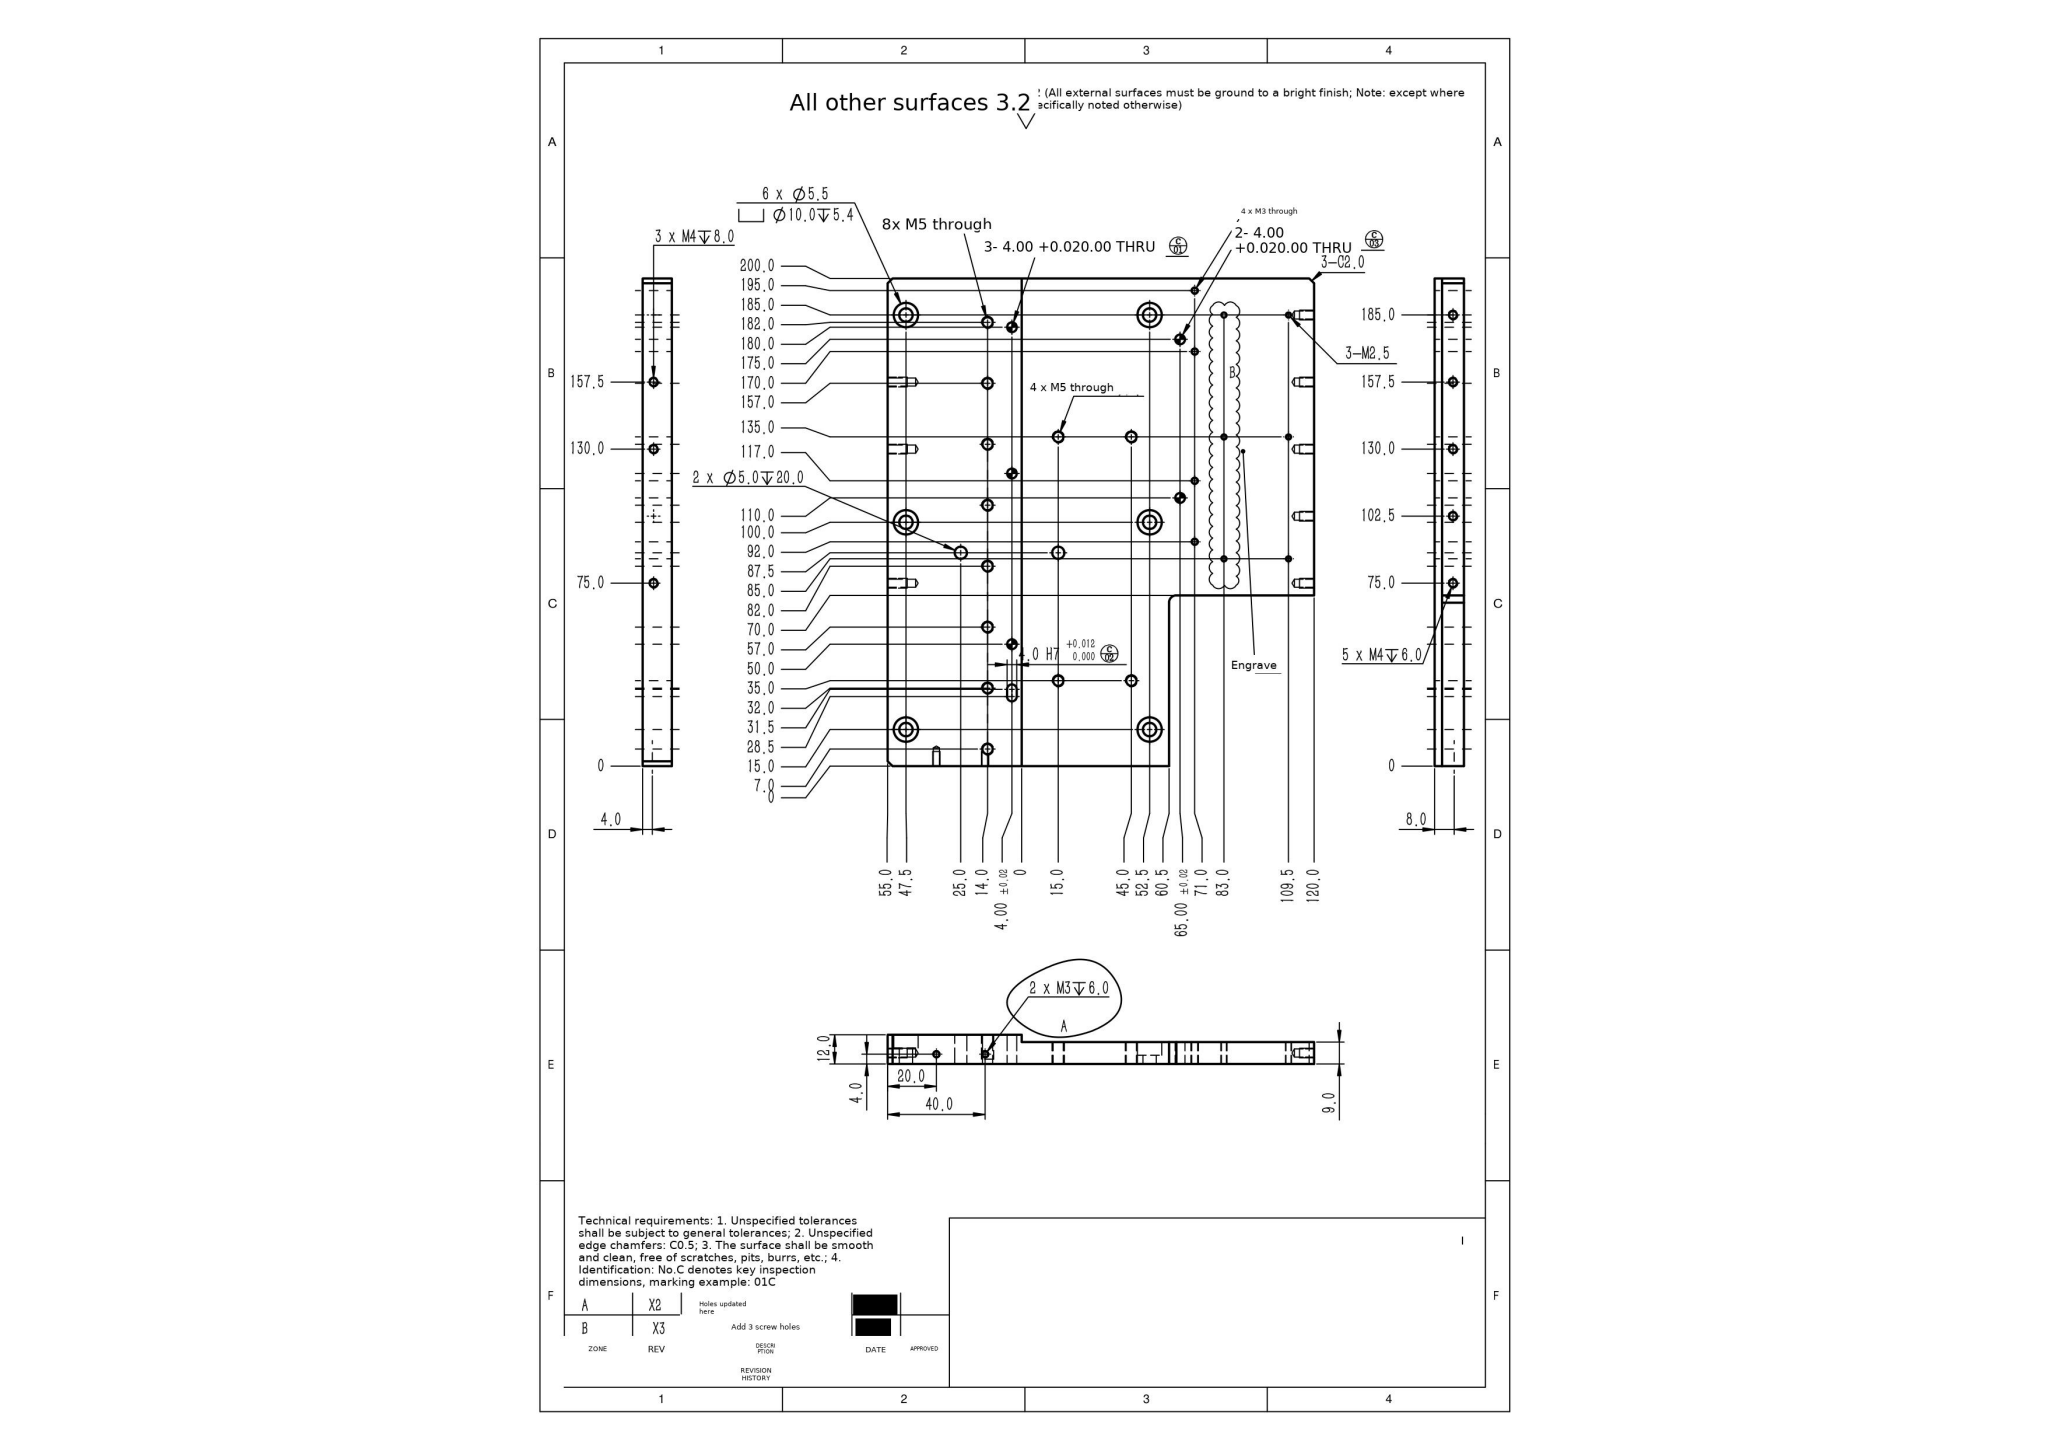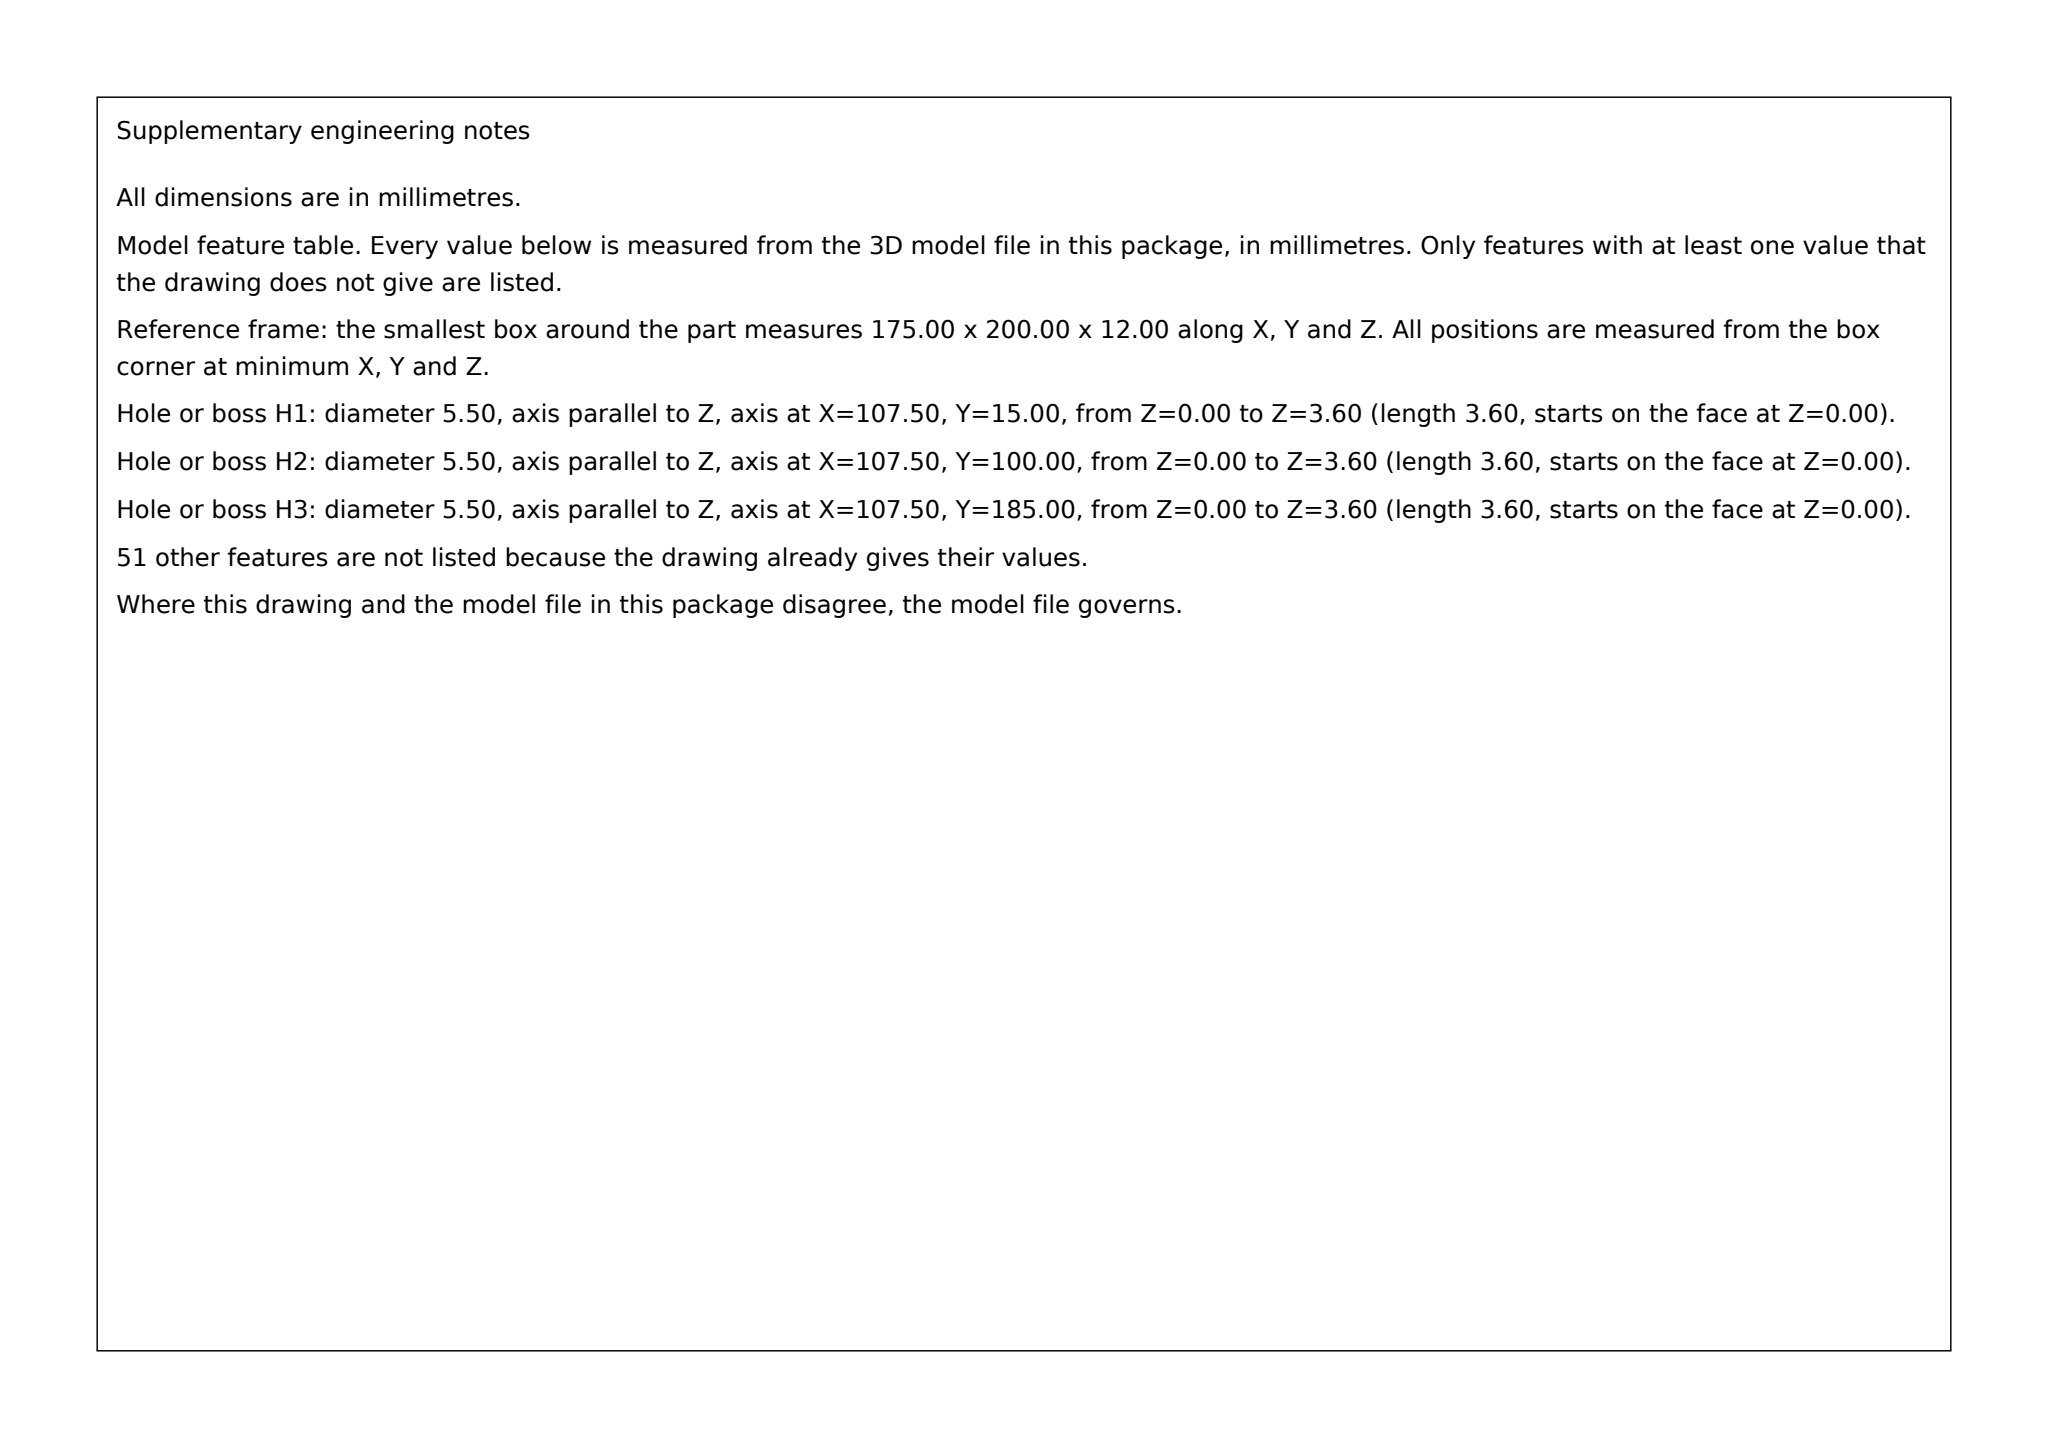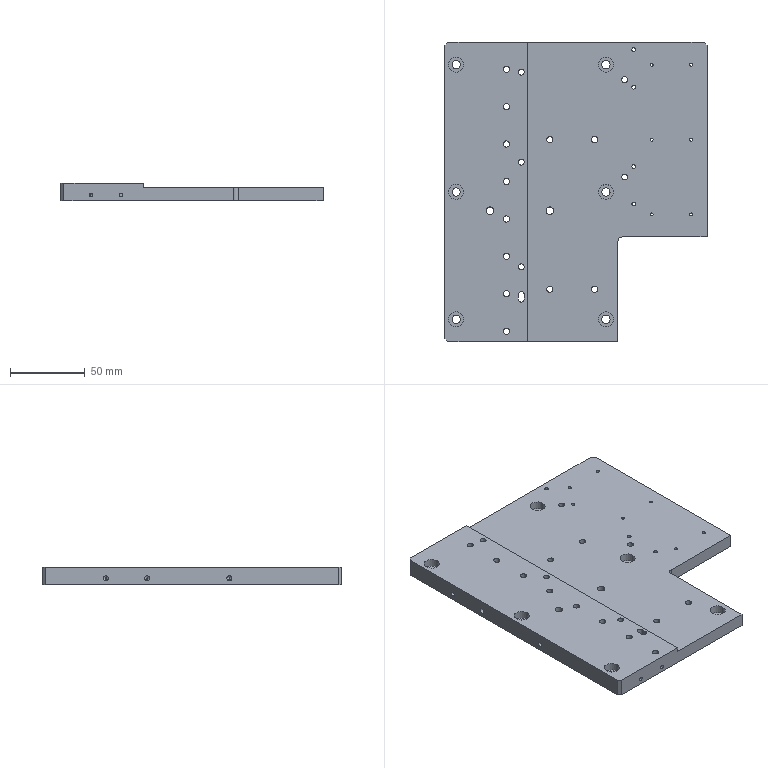Part | SolidWorks | mm | 1 solid | 145 faces | box 175 x 200 x 12 mm | volume 302897 mm3 | cylinder 105 | plane 21 | cone 19 | commonest cylinder face diameters 4.2 x24 3.3 x16 2.05 x12 2.5 x12 4 x12 10 x12 5.5 x12 5 x4
build123d program:
from build123d import *

# Parameters (mm, degrees)
SKETCH1_W                                       = 100
SKETCH1_H                                       = 150
BOSS_EXTRUDE1_DEPTH                             = 12
SKETCH2_W                                       = 60
SKETCH2_H                                       = 150
CUT_EXTRUDE1_DEPTH                              = 3
M5_TAPPED_HOLE2_D                               = 4.2
F_5_0_5_DIAMETER_HOLE1_D                        = 5
F_5_0_5_DIAMETER_HOLE1_DEPTH                    = 20
F_5_0_5_DIAMETER_HOLE1_TIP                      = 1.502
LPATTERN1_COUNT                                 = 6
LPATTERN1_PITCH                                 = 25
F_4_0_4_DIAMETER_HOLE1_D                        = 4
MOVE_FACE1_BY                                   = 15
MOVE_FACE2_BY                                   = 15
MOVE_FACE3_BY                                   = 50
M5_HEX_SOCKET_HEAD_CAP_SCREW_CBORE4_D           = 5.5
M5_HEX_SOCKET_HEAD_CAP_SCREW_CBORE4_CBORE_D     = 10
M5_HEX_SOCKET_HEAD_CAP_SCREW_CBORE4_CBORE_DEPTH = 5.4
M5_HEX_SOCKET_HEAD_CAP_SCREW_CBORE5_D           = 5.5
M5_HEX_SOCKET_HEAD_CAP_SCREW_CBORE5_CBORE_D     = 10
M5_HEX_SOCKET_HEAD_CAP_SCREW_CBORE5_CBORE_DEPTH = 5.4
CHAMFER1_SIZE                                   = 2
SKETCH23_R                                      = 2
CUT_EXTRUDE3_DEPTH                              = 232.017
SKETCH24_R                                      = 2
CUT_EXTRUDE4_DEPTH                              = 231.881
M3_TAPPED_HOLE1_D                               = 2.5
SKETCH27_W                                      = 9
SKETCH27_H                                      = 140
BOSS_EXTRUDE2_DEPTH                             = 45
M3_TAPPED_HOLE2_D                               = 2.5
M2_5_TAPPED_HOLE1_D                             = 2.05
FILLET1_R                                       = 3
M4_TAPPED_HOLE3_D                               = 3.3
M4_TAPPED_HOLE3_DEPTH                           = 8.1
M4_TAPPED_HOLE3_TIP                             = 0.9914
CHAMFER2_SIZE                                   = 2
M4_TAPPED_HOLE4_D                               = 3.3
M4_TAPPED_HOLE4_DEPTH                           = 11.5
M4_TAPPED_HOLE4_TIP                             = 0.9914
SKETCH40_W                                      = 30
SKETCH40_H                                      = 60
CUT_EXTRUDE5_DEPTH                              = 9
SKETCH41_W                                      = 59.5
SKETCH41_H                                      = 10
CUT_EXTRUDE6_DEPTH                              = 9
M5_TAPPED_HOLE3_D                               = 4.2
M5_TAPPED_HOLE3_DEPTH                           = 14
M5_TAPPED_HOLE3_TIP                             = 1.262
M3_TAPPED_HOLE3_D                               = 2.5
M3_TAPPED_HOLE3_DEPTH                           = 7.5
M3_TAPPED_HOLE3_TIP                             = 0.7511
LPATTERN3_COUNT                                 = 2
LPATTERN3_PITCH                                 = 26.5
FILLET2_R                                       = 3


with BuildPart() as part:
    # Sketch1 → Boss-Extrude1 (new body)
    with BuildSketch(Plane.XY):
        with Locations((50, 75)):
            Rectangle(SKETCH1_W, SKETCH1_H)
    extrude(amount=BOSS_EXTRUDE1_DEPTH)

    # Sketch2 → Cut-Extrude1 (cut)
    with BuildSketch(Plane.XY.offset(12)):
        with Locations((70, 75)):
            Rectangle(SKETCH2_W, SKETCH2_H)
    extrude(amount=-CUT_EXTRUDE1_DEPTH, mode=Mode.SUBTRACT)

    # Sketch3_2 → M5 Tapped Hole1 (revolve, cut)
    with BuildSketch(Plane(origin=(26, 132, 12), x_dir=(0, -1, 0), z_dir=(1, 0, 0))):
        Polygon((0, 0), (0, 15.262), (2.1, 14), (2.1, 0), align=None)
    m5_tapped_hole1 = revolve(axis=Axis((26, 132, 18.35), (0, 0, -1)), mode=Mode.SUBTRACT)

    # M5 Tapped Hole2 (through all)
    with Locations(Plane(origin=(0, 0, 0), x_dir=(-1, 0, 0), z_dir=(0, 0, -1))):
        with Locations((-85, 35), (-55, 35), (-85, 135), (-55, 135)):
            Hole(M5_TAPPED_HOLE2_D / 2)

    # 5.0 _5_ Diameter Hole1
    with Locations(Plane(origin=(0, 0, 0), x_dir=(-1, 0, 0), z_dir=(0, 0, -1))):
        with Locations((-55, 87.5), (-15, 87.5)):
            Hole(F_5_0_5_DIAMETER_HOLE1_D / 2, depth=F_5_0_5_DIAMETER_HOLE1_DEPTH)
            with Locations((0, 0, -(F_5_0_5_DIAMETER_HOLE1_DEPTH + F_5_0_5_DIAMETER_HOLE1_TIP / 2))):  # 118° drill point
                Cone(0, F_5_0_5_DIAMETER_HOLE1_D / 2, F_5_0_5_DIAMETER_HOLE1_TIP, mode=Mode.SUBTRACT)

    # LPattern1: M5 Tapped Hole1 ×6
    with Locations(*[(0, -i * LPATTERN1_PITCH, 0) for i in range(1, LPATTERN1_COUNT)]):
        add(m5_tapped_hole1, mode=Mode.SUBTRACT)

    # 4.0 _4_ Diameter Hole1 (through all)
    with Locations(Plane(origin=(-0.2203, 3.564, 12), x_dir=(1, 0, 0), z_dir=(0, 0, 1))):
        with Locations((36.22, 116.436), (36.22, 46.436)):
            Hole(F_4_0_4_DIAMETER_HOLE1_D / 2)

    # Move Face1: a face moved outward by 15.0
    extrude(part.faces().sort_by_distance((100, 75, 4.5))[0], amount=MOVE_FACE1_BY, dir=(1, 0, 0))

    # Move Face2: a face moved outward by 15.0
    extrude(part.faces().sort_by_distance((0, 75, 6))[0], amount=MOVE_FACE2_BY, dir=(-1, 0, 0))

    # Move Face3: a face moved outward by 50.0
    extrude(part.faces().sort_by_distance((45.365, 150, 5.242))[0], amount=MOVE_FACE3_BY, dir=(0, 1, 0))

    # M5 Hex Socket Head Cap Screw CBORE4 (through all)
    with Locations(Plane.XY.offset(9)):
        with Locations((92.5, 185), (92.5, 100), (92.5, 15)):
            CounterBoreHole(M5_HEX_SOCKET_HEAD_CAP_SCREW_CBORE4_D / 2, M5_HEX_SOCKET_HEAD_CAP_SCREW_CBORE4_CBORE_D / 2, M5_HEX_SOCKET_HEAD_CAP_SCREW_CBORE4_CBORE_DEPTH)

    # M5 Hex Socket Head Cap Screw CBORE5 (through all)
    with Locations(Plane.XY.offset(12)):
        with Locations((-7.5, 185), (-7.5, 100), (-7.5, 15)):
            CounterBoreHole(M5_HEX_SOCKET_HEAD_CAP_SCREW_CBORE5_D / 2, M5_HEX_SOCKET_HEAD_CAP_SCREW_CBORE5_CBORE_D / 2, M5_HEX_SOCKET_HEAD_CAP_SCREW_CBORE5_CBORE_DEPTH)

    # Chamfer1
    chamfer1_edges = [part.edges().sort_by_distance(p)[0] for p in [
        (-15, 200, 6),
        (-15, 0, 6),
    ]]
    chamfer(chamfer1_edges, length=CHAMFER1_SIZE)

    # Sketch23 → Cut-Extrude3 (cut, through all)
    with BuildSketch(Plane.XY.offset(12)):
        with Locations((36, 180)):
            Circle(SKETCH23_R)
        with BuildLine():
            Line((38, 31.5), (38, 28.5))
            ThreePointArc((38, 28.5), (36, 26.5), (34, 28.5))
            Line((34, 28.5), (34, 31.5))
            ThreePointArc((34, 31.5), (36, 33.5), (38, 31.5))
        make_face()
    extrude(amount=-CUT_EXTRUDE3_DEPTH, mode=Mode.SUBTRACT)

    # Sketch24 → Cut-Extrude4 (cut, through all)
    with BuildSketch(Plane.XY.offset(9)):
        with Locations((105, 175)):
            Circle(SKETCH24_R)
        with Locations((105, 110)):
            Circle(SKETCH24_R)
    extrude(amount=-CUT_EXTRUDE4_DEPTH, mode=Mode.SUBTRACT)

    # M3 Tapped Hole1 (through all)
    with Locations(Plane.XY.offset(9)):
        with Locations((111, 195), (111, 117)):
            Hole(M3_TAPPED_HOLE1_D / 2)

    # Sketch27 → Boss-Extrude2 (add)
    with BuildSketch(Plane(origin=(115, 0, 0), x_dir=(0, 0, -1), z_dir=(1, 0, 0))):
        with Locations((-4.5, 130)):
            Rectangle(SKETCH27_W, SKETCH27_H)
    extrude(amount=BOSS_EXTRUDE2_DEPTH)

    # M3 Tapped Hole2 (through all)
    with Locations(Plane.XY.offset(9)):
        with Locations((111, 170), (111, 92)):
            Hole(M3_TAPPED_HOLE2_D / 2)

    # M2.5 Tapped Hole1 (through all)
    with Locations(Plane.XY.offset(9)):
        with Locations((149.5, 185), (149.5, 85), (149.5, 135)):
            m2_5_tapped_hole1 = Hole(M2_5_TAPPED_HOLE1_D / 2)

    # Fillet1
    fillet1_edges = [part.edges().sort_by_distance(p)[0] for p in [
        (115, 60, 4.5),
    ]]
    fillet(fillet1_edges, radius=FILLET1_R)

    # M4 Tapped Hole3
    with Locations(Plane(origin=(160, 0, 0), x_dir=(0, 0, -1), z_dir=(1, 0, 0))):
        with Locations((-4.5, 185), (-4.5, 130), (-4.5, 75), (-4.5, 157.5), (-4.5, 102.5)):
            Hole(M4_TAPPED_HOLE3_D / 2, depth=M4_TAPPED_HOLE3_DEPTH)
            with Locations((0, 0, -(M4_TAPPED_HOLE3_DEPTH + M4_TAPPED_HOLE3_TIP / 2))):  # 118° drill point
                Cone(0, M4_TAPPED_HOLE3_D / 2, M4_TAPPED_HOLE3_TIP, mode=Mode.SUBTRACT)

    # Chamfer2
    chamfer2_edges = [part.edges().sort_by_distance(p)[0] for p in [
        (160, 200, 4.5),
        (160, 60, 4.5),
        (115, 0, 4.5),
    ]]
    chamfer(chamfer2_edges, length=CHAMFER2_SIZE)

    # M4 Tapped Hole4
    with Locations(Plane.ZY.offset(15)):
        with Locations((4.5, 157.5), (4.5, 130), (4.5, 75)):
            Hole(M4_TAPPED_HOLE4_D / 2, depth=M4_TAPPED_HOLE4_DEPTH)
            with Locations((0, 0, -(M4_TAPPED_HOLE4_DEPTH + M4_TAPPED_HOLE4_TIP / 2))):  # 118° drill point
                Cone(0, M4_TAPPED_HOLE4_D / 2, M4_TAPPED_HOLE4_TIP, mode=Mode.SUBTRACT)

    # Sketch40 → Cut-Extrude5 (cut)
    with BuildSketch(Plane.XY.offset(9)):
        with Locations((115.5, 30)):
            Rectangle(SKETCH40_W, SKETCH40_H)
    extrude(amount=-CUT_EXTRUDE5_DEPTH, mode=Mode.SUBTRACT)

    # Sketch41 → Cut-Extrude6 (cut)
    with BuildSketch(Plane.XY.offset(9)):
        with Locations((130.25, 65)):
            Rectangle(SKETCH41_W, SKETCH41_H)
    extrude(amount=-CUT_EXTRUDE6_DEPTH, mode=Mode.SUBTRACT)

    # M5 Tapped Hole3
    with Locations(Plane.XY.offset(12)):
        with Locations((26, 182), (26, 157)):
            Hole(M5_TAPPED_HOLE3_D / 2, depth=M5_TAPPED_HOLE3_DEPTH)
            with Locations((0, 0, -(M5_TAPPED_HOLE3_DEPTH + M5_TAPPED_HOLE3_TIP / 2))):  # 118° drill point
                Cone(0, M5_TAPPED_HOLE3_D / 2, M5_TAPPED_HOLE3_TIP, mode=Mode.SUBTRACT)

    # M3 Tapped Hole3
    with Locations(Plane(origin=(0, 0, 0), x_dir=(-1, 0, 0), z_dir=(0, -1, 0))):
        with Locations((-5, -4), (-25, -4)):
            Hole(M3_TAPPED_HOLE3_D / 2, depth=M3_TAPPED_HOLE3_DEPTH)
            with Locations((0, 0, -(M3_TAPPED_HOLE3_DEPTH + M3_TAPPED_HOLE3_TIP / 2))):  # 118° drill point
                Cone(0, M3_TAPPED_HOLE3_D / 2, M3_TAPPED_HOLE3_TIP, mode=Mode.SUBTRACT)

    # LPattern3: M2.5 Tapped Hole1 ×2
    with Locations(*[(-i * LPATTERN3_PITCH, 0, 0) for i in range(1, LPATTERN3_COUNT)]):
        add(m2_5_tapped_hole1, mode=Mode.SUBTRACT)

    # Fillet2
    fillet2_edges = [part.edges().sort_by_distance(p)[0] for p in [
        (100.5, 70, 4.5),
    ]]
    fillet(fillet2_edges, radius=FILLET2_R)


solid = part.part